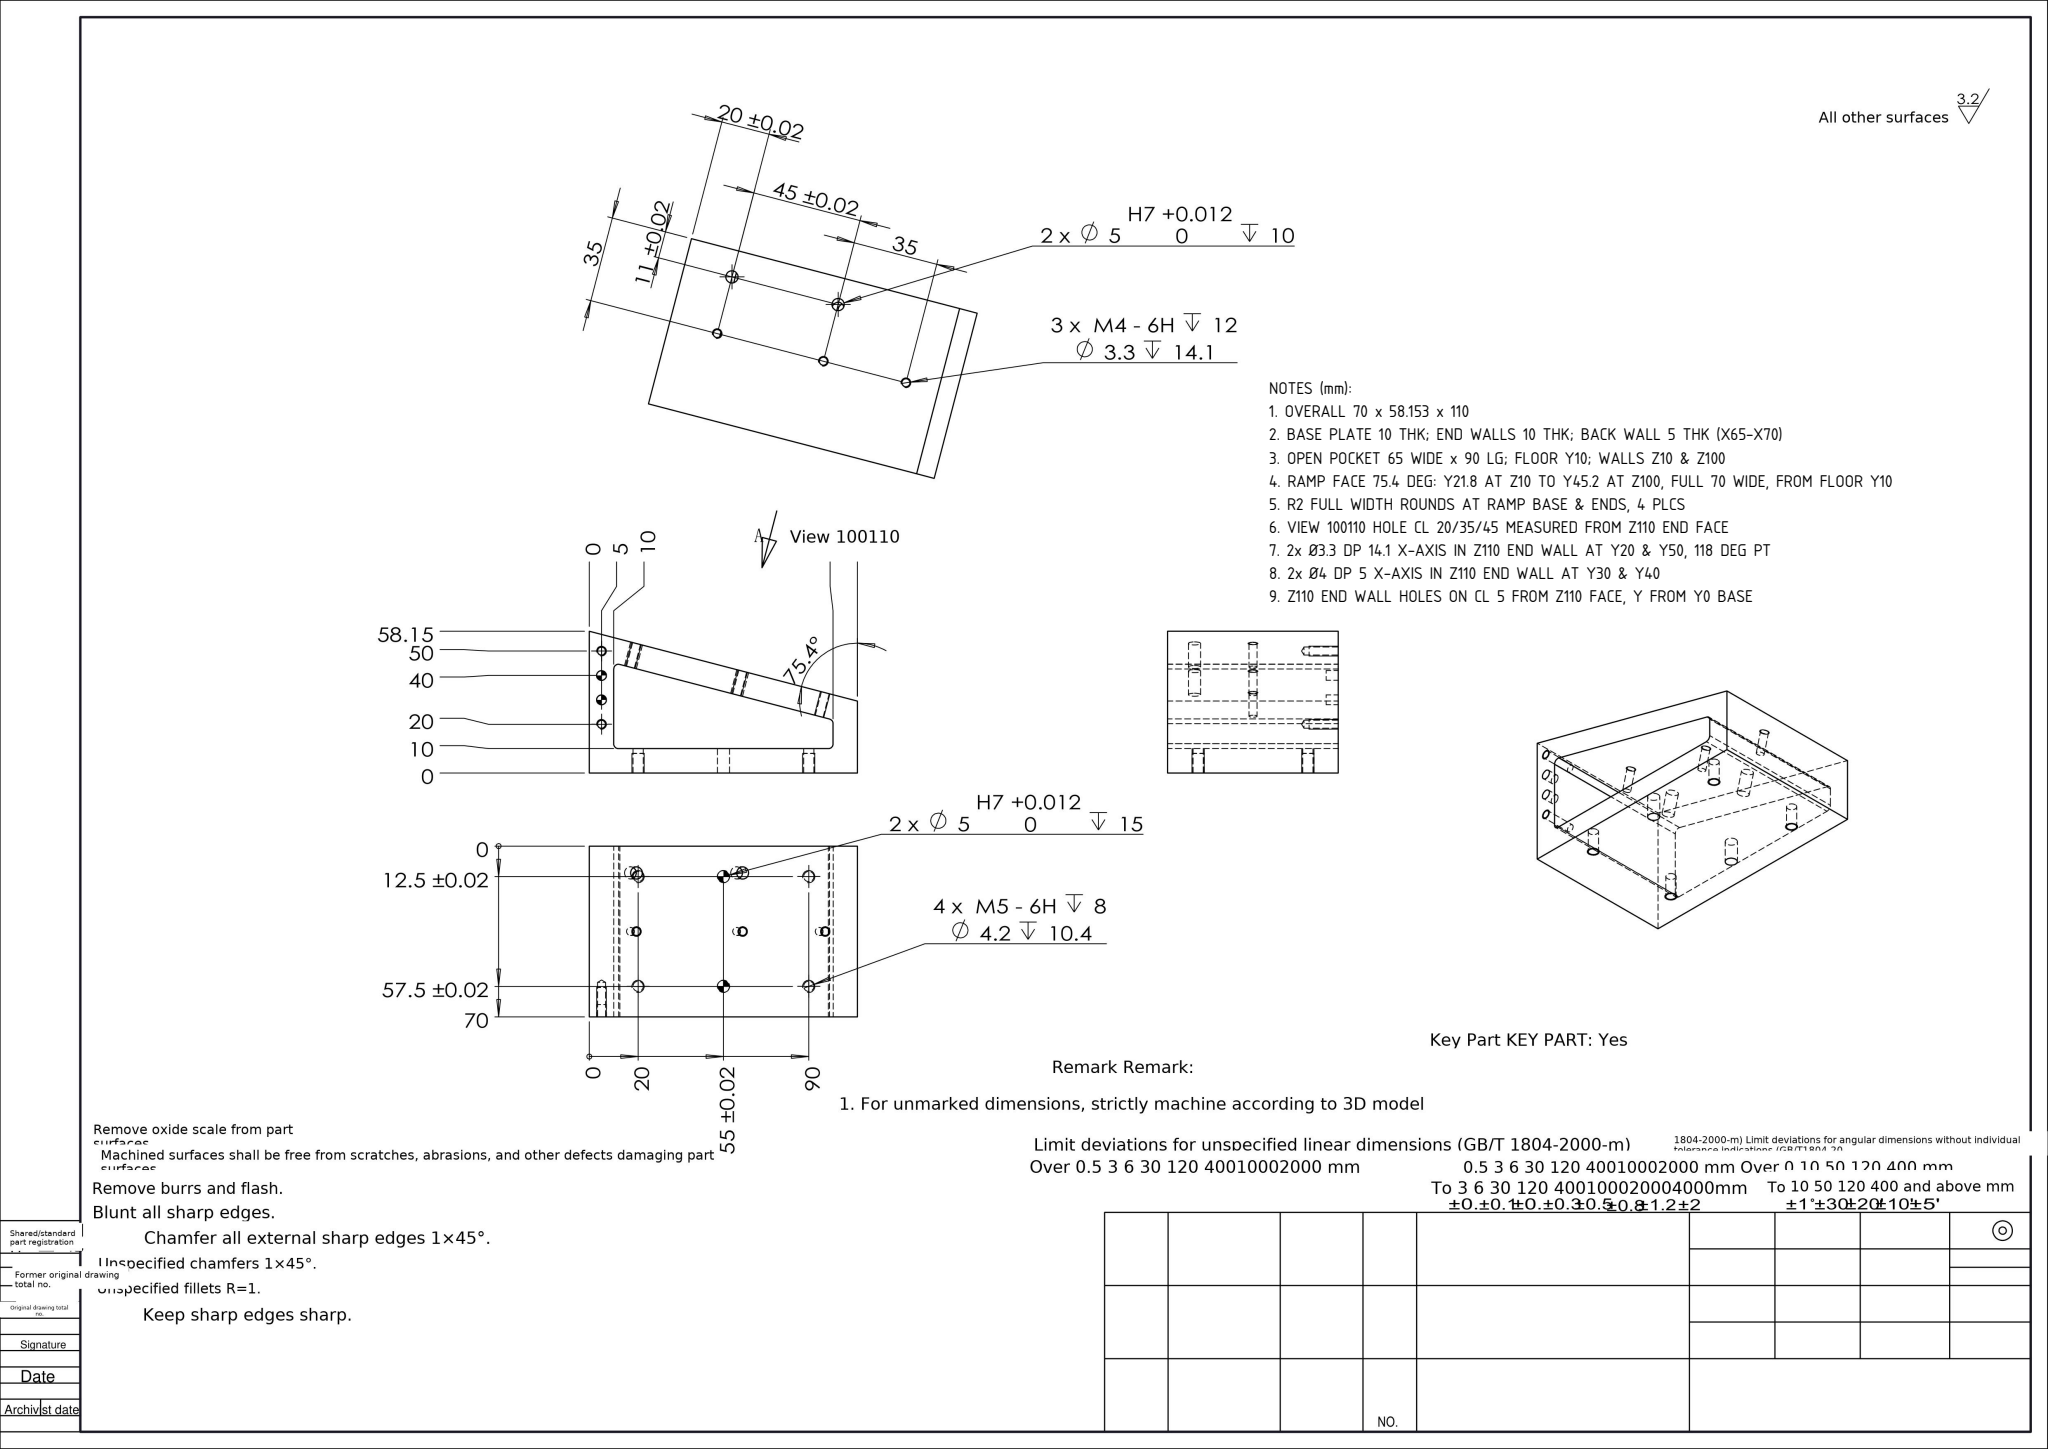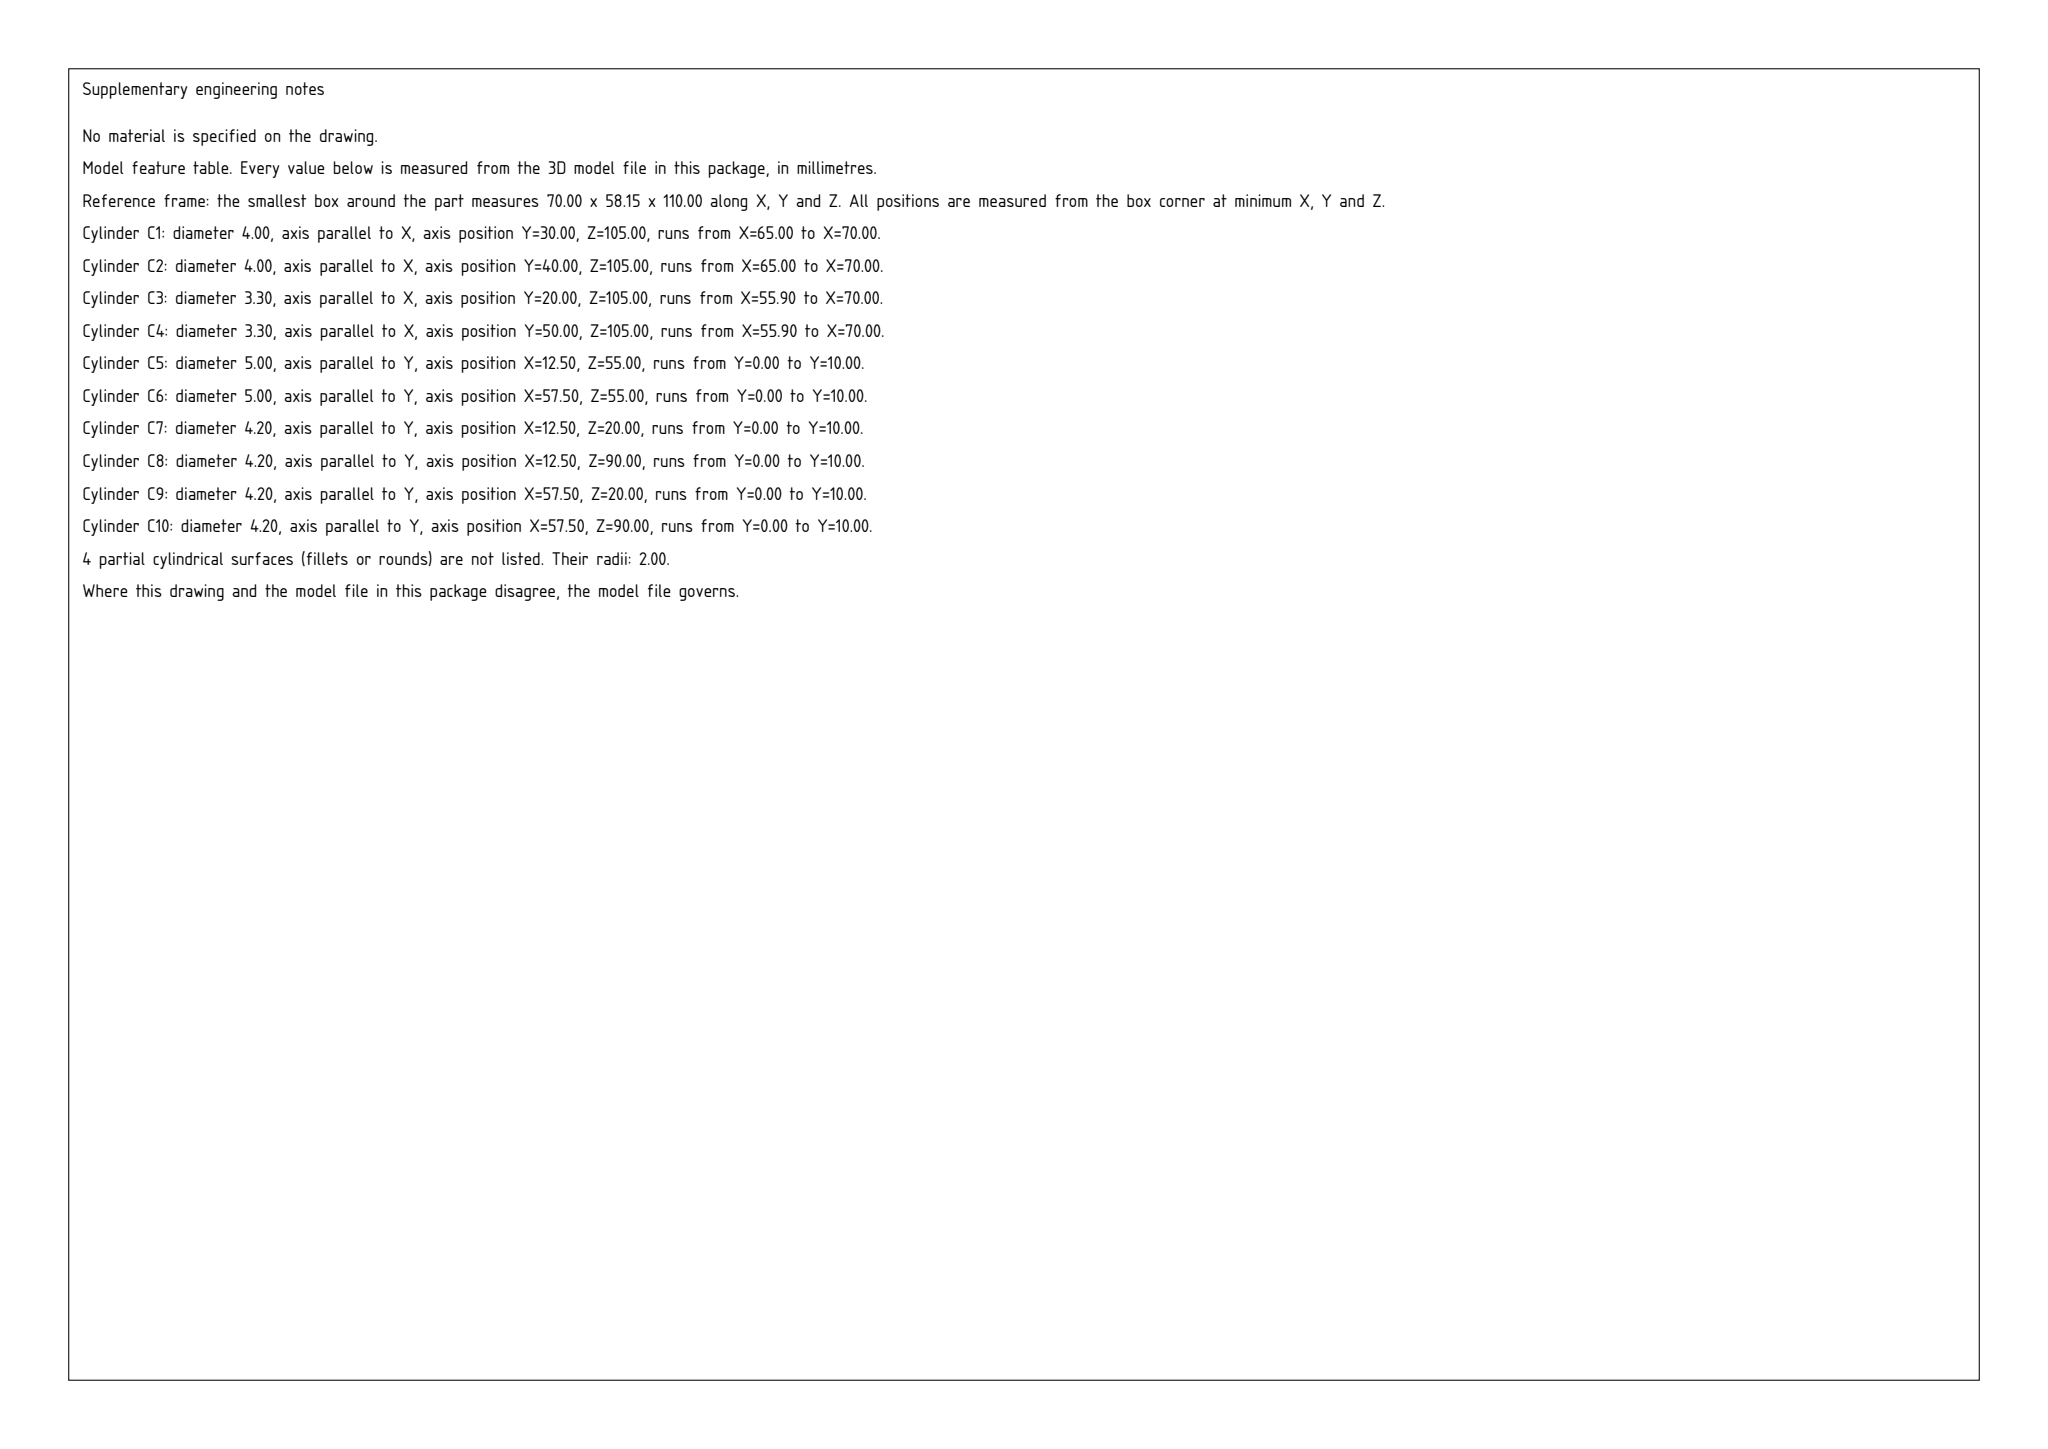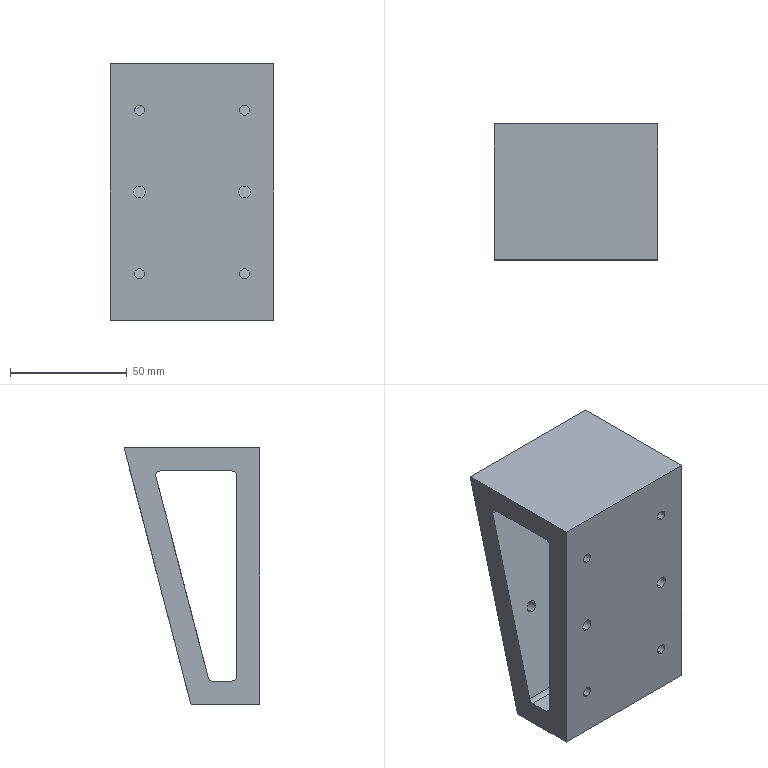Part | SolidWorks | mm | 1 solid | 50 faces | box 70 x 58.15 x 110 mm | volume 187750 mm3 | cylinder 34 | plane 12 | cone 4 | commonest cylinder face diameters 3.3 x10 5 x8 4.2 x8 4 x8
Drawing notes:
OVERALL 70 x 58.153 x 110 | from the solid: bbox_xyz 70.0 x 58.153 x 110.0
BASE PLATE 10 THK; END WALLS 10 THK; BACK WALL 5 THK (X65-X70) | from the solid: axis_planes y=0/10, z=0/10 & z=100/110, x=65/70
OPEN POCKET 65 WIDE x 90 LG; FLOOR Y10; WALLS Z10 & Z100 | from the solid: planes x=0..65, z=10 & 100, floor y=10
RAMP FACE 75.4 DEG: Y21.8 AT Z10 TO Y45.2 AT Z100, FULL 70 WIDE, FROM FLOOR Y10 | from the solid: R2 Ø4 x-axis rounds at (12,12),(20.23,12),(12,98),(42.63,98); tangent face
R2 FULL WIDTH ROUNDS AT RAMP BASE & ENDS, 4 PLCS | from the solid: 4x cyl Ø4.0 axis x, len 70 at (12,12),(20.23,12),(12,98),(42.63,98)
VIEW 100110 HOLE CL 20/35/45 MEASURED FROM Z110 END FACE | from the solid: holes on ramp face at z=90.65, 47.1, 13.23 = 20/35/45 x cos14.6
2x Ø3.3 DP 14.1 X-AXIS IN Z110 END WALL AT Y20 & Y50, 118 DEG PT | from the solid: cyl Ø3.3 axis x at (y20,z105) & (y50,z105) len 14.1; cone 118 deg
2x Ø4 DP 5 X-AXIS IN Z110 END WALL AT Y30 & Y40 | from the solid: cyl Ø4.0 axis x at (y30,z105) & (y40,z105) len 5.0
Z110 END WALL HOLES ON CL 5 FROM Z110 FACE, Y FROM Y0 BASE | from the solid: x-axis holes at z=105.0 with end face plane z=110